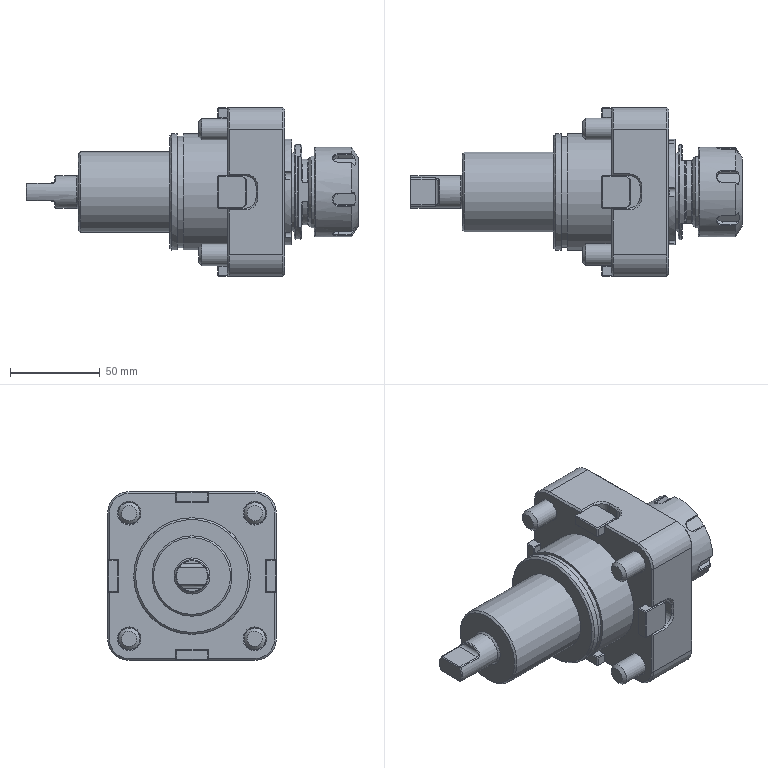Assembly | NX | mm | 6 component files | 6 solids | 423 faces | box 185 x 94 x 94 mm | volume 513863 mm3 | plane 272 | cone 61 | cylinder 58 | spline 22 | torus 10 | commonest cylinder face diameters 12 x12 6.4 x6 24 x5 5 x5 18 x4 12.2 x4 18.4 x4 36.6 x2
Bill of materials:
unnamed part 1 | 4 |  | Headed pin or screw-like solid: a short cylindrical head with rounded outer edge and a polygonal (hex-like) socket recess in its end face, plus a longer plain cylindrical shank of smaller diameter ending in a chamfered tip.
unnamed part 2 | 1 |  | Thick annular ring or nut-like body with a large central through-bore, a chamfered front end, a stepped or recessed front face, and several (about 6-7) rounded-end slots spaced around its outer surface, open toward the chamfered end.
unnamed part 3 | 1 |  | Flanged, stepped cylindrical housing: a square plate flange with rounded corners and four corner through-holes, a short front cylindrical boss with a central bore and annular grooves/rings, and a longer stepped cylindrical rear body ending in a small rectangular/keyed projection. Small tab or clip features stick out at the sides of the flange.
Mates:
1. fix | 12_01_Body 1 component
2. touch align | 12_02_Nut_ER32UM 1 face | 12_01_Body 1 face
3. concentric | 12_03_Screw_M12x35_DIN912 4 edge | 12_01_Body 1 edge
4. bond | 12_01_Body 1 component | assembly component
5. bond | 12_01_Body 1 component | assembly component
6. bond | 12_03_Screw_M12x35_DIN912 4 component | assembly component
7. bond | 12_03_Screw_M12x35_DIN912 3 component | assembly component
8. bond | 12_03_Screw_M12x35_DIN912 2 component | assembly component
9. bond | 12_03_Screw_M12x35_DIN912 1 component | assembly component
10. linear | assembly datumaxis | assembly datumaxis | assembly cartesiancoordinatesystem | assembly cartesiancoordinatesystem | assembly cartesiancoordinatesystem | assembly cartesiancoordinatesystem